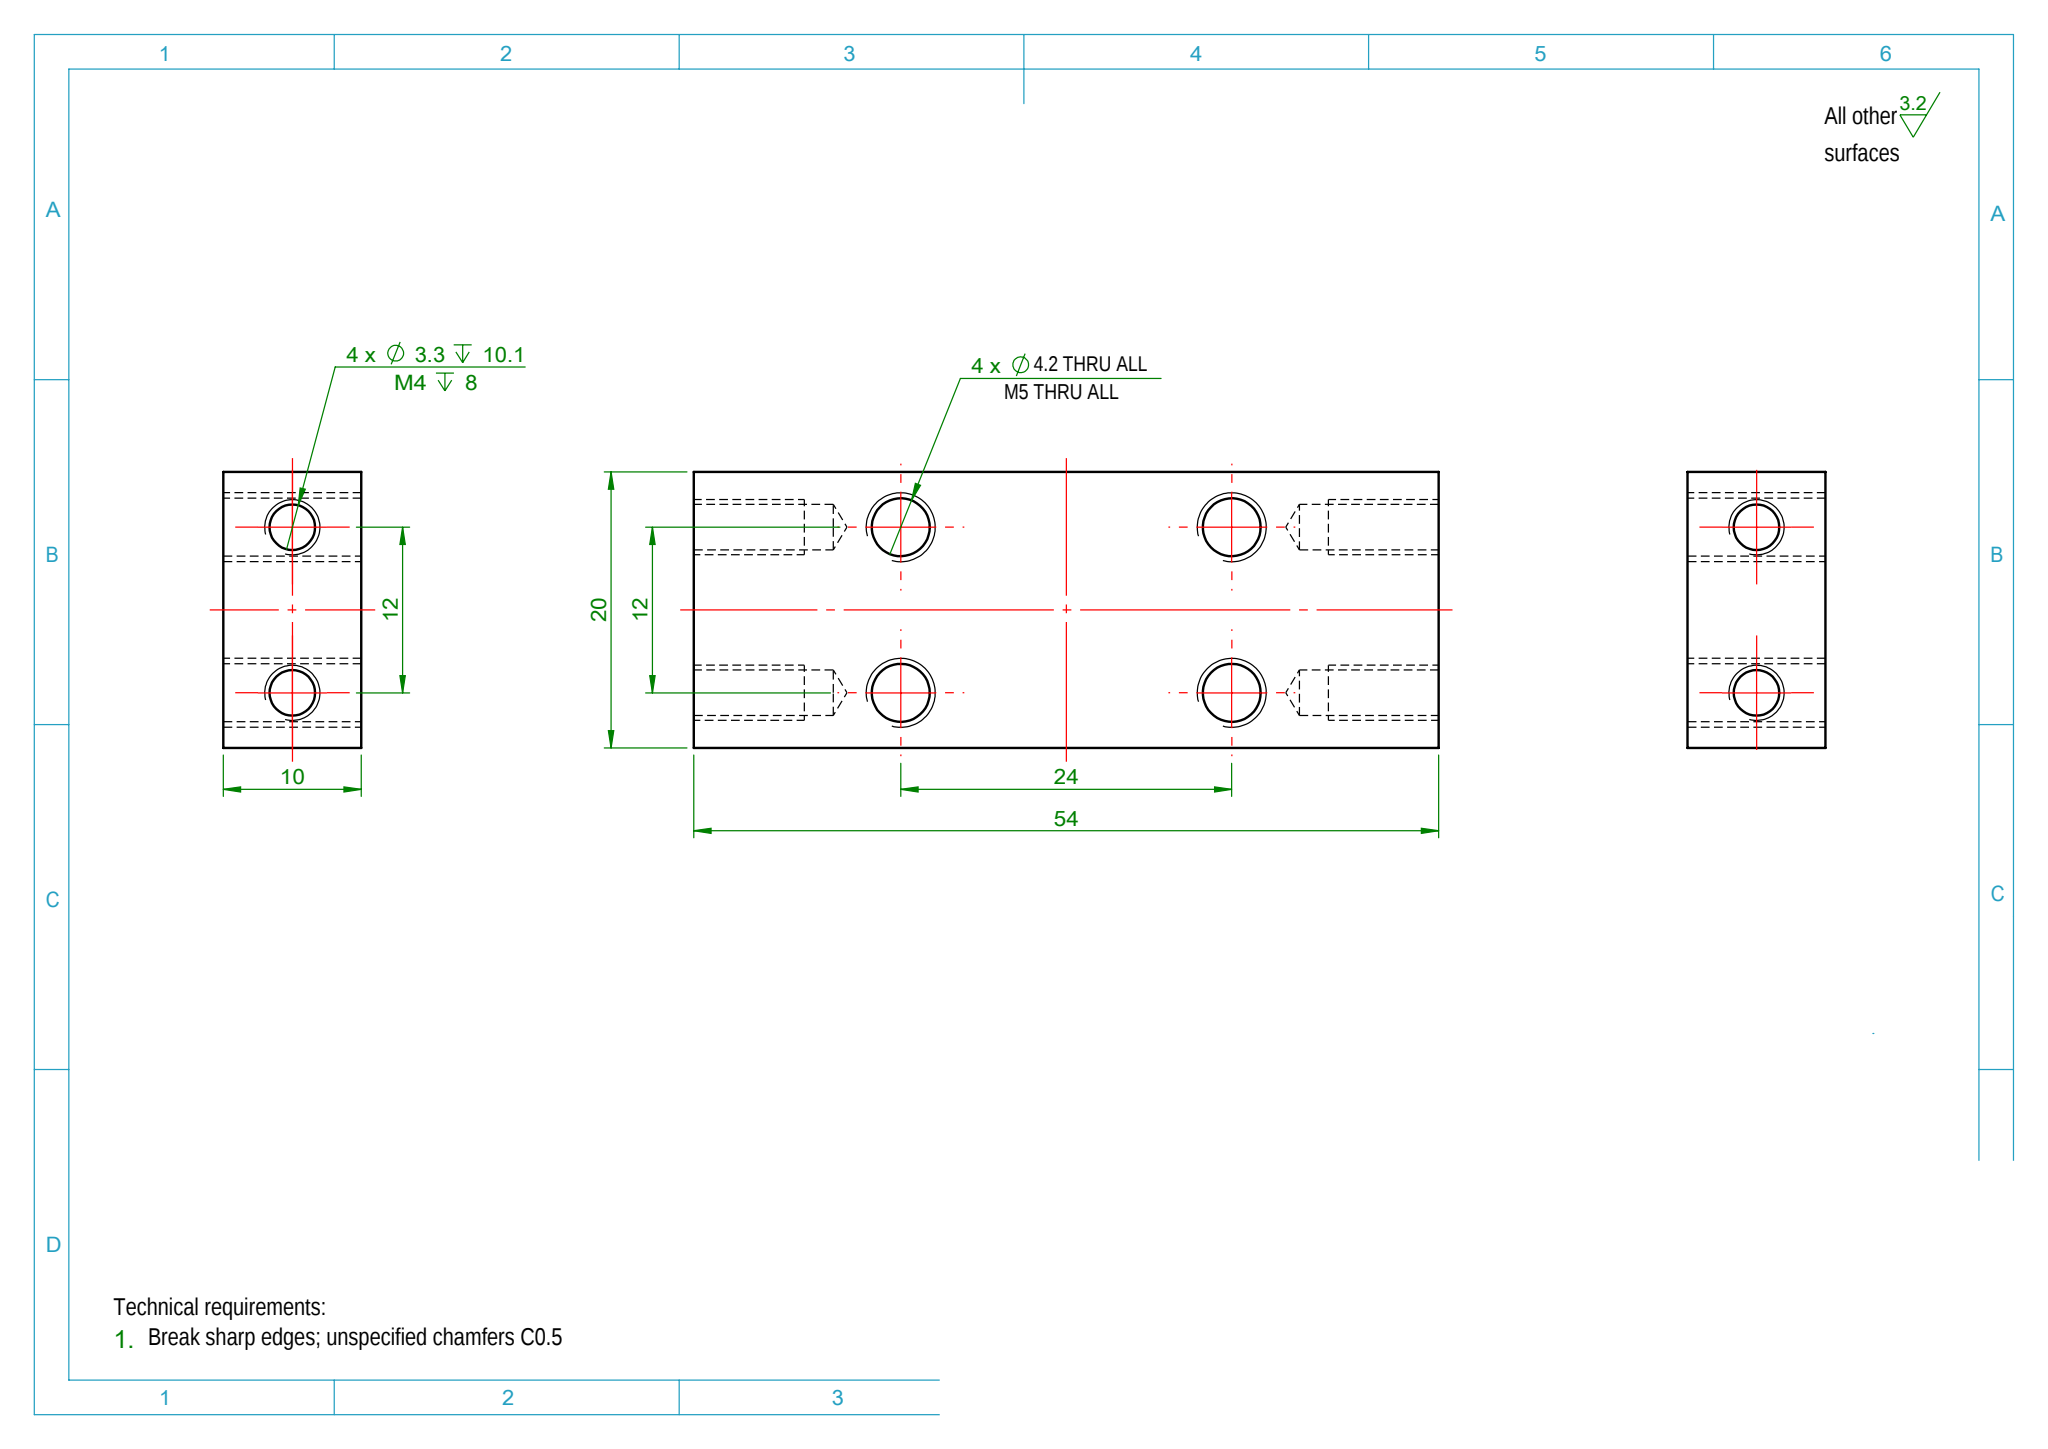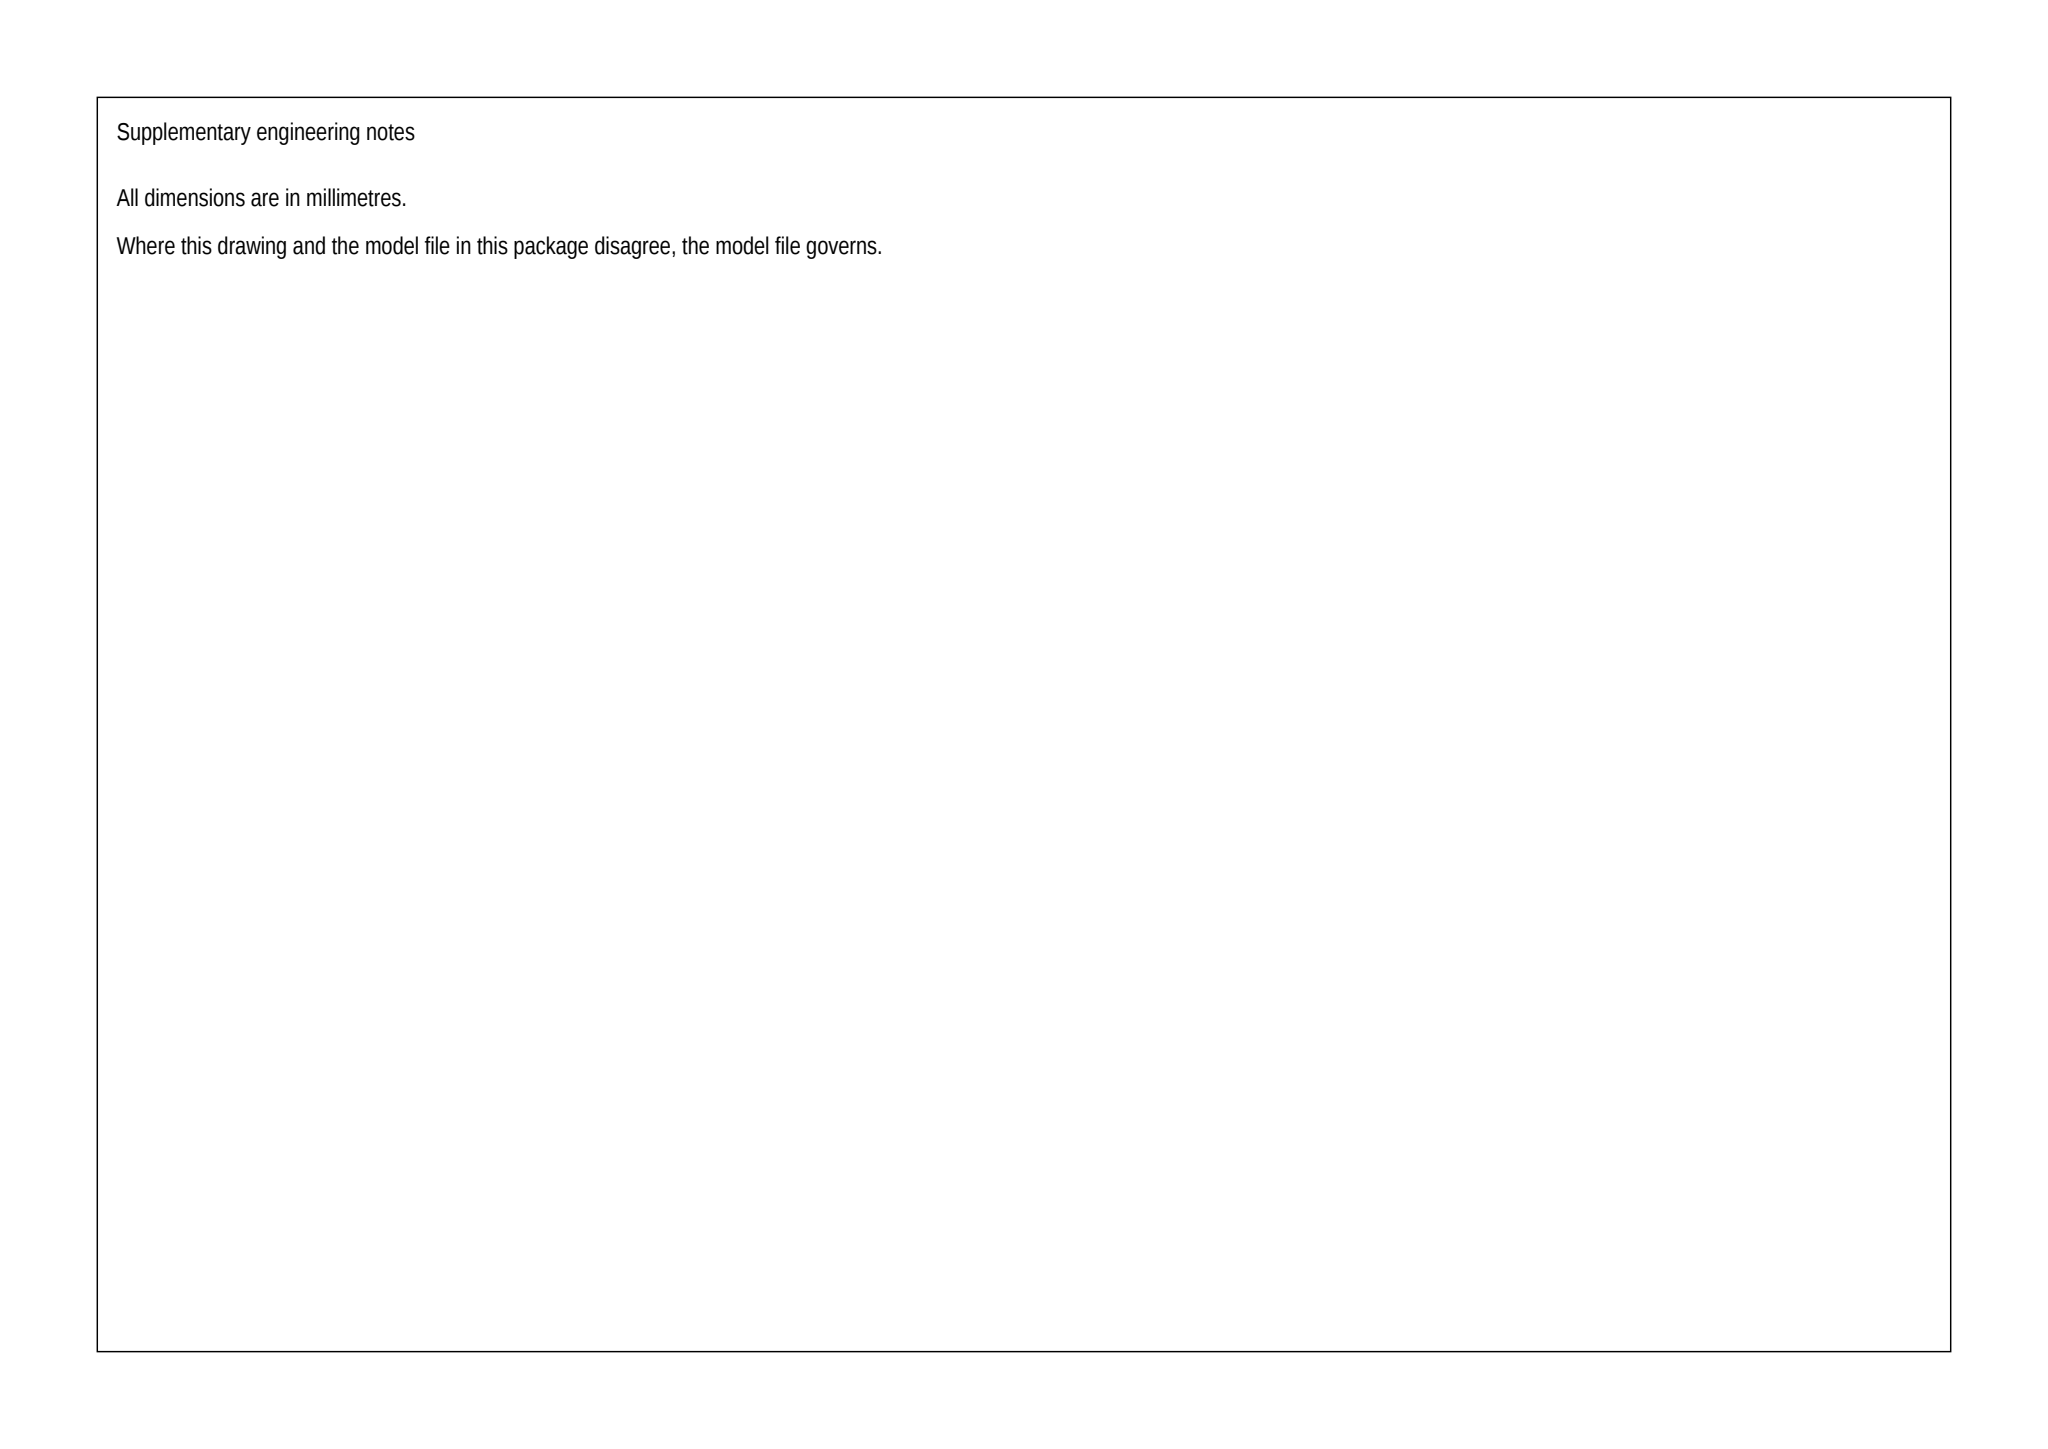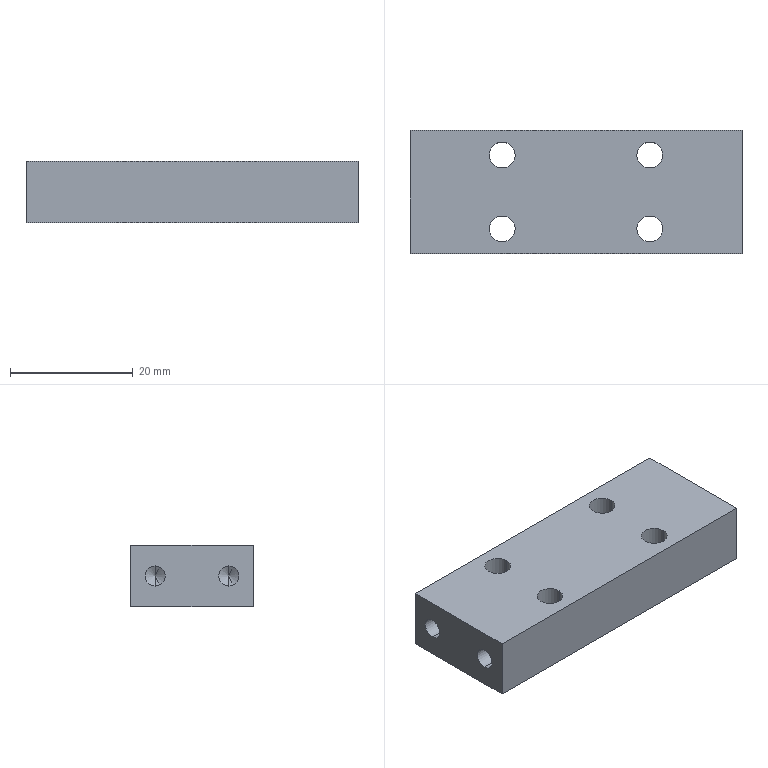Part | SolidWorks | mm | 1 solid | 30 faces | box 54 x 20 x 10 mm | volume 9889 mm3 | cylinder 16 | cone 8 | plane 6 | commonest cylinder face diameters 4.2 x8 3.3 x8
Drawing notes:
4X Ø4.2 THRU (through 10 thk plate), vertical axes; hole centers at X=15 and X=39 from left end face and Y=4 and Y=16 from bottom long edge. | from the solid: cylinders dia 4.2, axis z, length 10.0 at (15,4),(15,16),(39,4),(39,16); bbox_xyz 54x20x10
All dimensions in millimeters (mm) unless otherwise stated. | from the solid: STEP model units stated as mm; bbox_xyz [54.0, 20.0, 10.0]
build123d program:
from build123d import *

# Parameters (mm, degrees)
SKETCH1_W                  = 54
SKETCH1_H                  = 20
BOSS_EXTRUDE1_DEPTH        = 10
M4_TAPPED_HOLE1_AT_2_COUNT = 2
M4_TAPPED_HOLE1_AT_2_PITCH = 12
M5_TAPPED_HOLE1_D          = 4.2


with BuildPart() as part:
    # Sketch1 → Boss-Extrude1 (new body)
    with BuildSketch(Plane.XY):
        Rectangle(SKETCH1_W, SKETCH1_H)
    extrude(amount=BOSS_EXTRUDE1_DEPTH)

    # Sketch3 → M4 Tapped Hole1 (revolve, cut)
    with BuildSketch(Plane(origin=(-27, 6, 5), x_dir=(0, 0, 1), z_dir=(0, 1, 0))):
        Polygon((0, 0), (0, 11.091), (1.65, 10.1), (1.65, 0), align=None)
    m4_tapped_hole1 = revolve(axis=Axis((-33.35, 6, 5), (1, 0, 0)), mode=Mode.SUBTRACT)

    # M4 Tapped Hole1 at 2: M4 Tapped Hole1 ×2
    with Locations(*[(0, -i * M4_TAPPED_HOLE1_AT_2_PITCH, 0) for i in range(1, M4_TAPPED_HOLE1_AT_2_COUNT)]):
        add(m4_tapped_hole1, mode=Mode.SUBTRACT)

    # Mirror1: M4 Tapped Hole1 across plane
    add(m4_tapped_hole1.mirror(Plane(origin=(0, 0, 0), x_dir=(0, 0, 1), z_dir=(1, 0, 0))), mode=Mode.SUBTRACT)

    # Mirror1 copy 1 sketch → Mirror1 copy 1 (revolve, cut)
    with BuildSketch(Plane(origin=(27, -6, 5), x_dir=(0, 0, 1), z_dir=(0, 1, 0))):
        Polygon((0, 0), (0, -11.091), (1.65, -10.1), (1.65, 0), align=None)
    revolve(axis=Axis((33.35, -6, 5), (1, 0, 0)), mode=Mode.SUBTRACT)

    # M5 Tapped Hole1 (through all)
    with Locations(Plane.XY.offset(10)):
        with Locations((-12, 6), (-12, -6), (12, 6), (12, -6)):
            Hole(M5_TAPPED_HOLE1_D / 2)


solid = part.part
STEP:
#1=CARTESIAN_POINT('',(-14.1,6.,0.));
#2=VERTEX_POINT('',#1);
#3=CARTESIAN_POINT('',(-9.9,6.,0.));
#4=VERTEX_POINT('',#3);
#5=CARTESIAN_POINT('',(-12.,6.,0.));
#6=DIRECTION('',(0.,0.,1.));
#7=DIRECTION('',(1.,0.,0.));
#8=AXIS2_PLACEMENT_3D('',#5,#6,#7);
#9=CIRCLE('',#8,2.1);
#10=EDGE_CURVE('',#2,#4,#9,.T.);
#11=ORIENTED_EDGE('',*,*,#10,.F.);
#12=CARTESIAN_POINT('',(-14.1,6.,10.));
#13=VERTEX_POINT('',#12);
#14=CARTESIAN_POINT('',(-14.1,6.,10.));
#15=DIRECTION('',(0.,0.,1.));
#16=VECTOR('',#15,1000.);
#17=LINE('',#14,#16);
#18=EDGE_CURVE('',#2,#13,#17,.T.);
#19=ORIENTED_EDGE('',*,*,#18,.T.);
#20=CARTESIAN_POINT('',(-9.9,6.,10.));
#21=VERTEX_POINT('',#20);
#22=CARTESIAN_POINT('',(-12.,6.,10.));
#23=DIRECTION('',(0.,0.,1.));
#24=DIRECTION('',(1.,0.,0.));
#25=AXIS2_PLACEMENT_3D('',#22,#23,#24);
#26=CIRCLE('',#25,2.1);
#27=EDGE_CURVE('',#13,#21,#26,.T.);
#28=ORIENTED_EDGE('',*,*,#27,.T.);
#29=CARTESIAN_POINT('',(-9.9,6.,10.));
#30=DIRECTION('',(0.,0.,1.));
#31=VECTOR('',#30,1000.);
#32=LINE('',#29,#31);
#33=EDGE_CURVE('',#4,#21,#32,.T.);
#34=ORIENTED_EDGE('',*,*,#33,.F.);
#35=EDGE_LOOP('',(#11,#19,#28,#34));
#36=FACE_OUTER_BOUND('',#35,.T.);
#37=CARTESIAN_POINT('',(-12.,6.,10.));
#38=DIRECTION('',(0.,0.,1.));
#39=DIRECTION('',(1.,0.,0.));
#40=AXIS2_PLACEMENT_3D('',#37,#38,#39);
#41=CYLINDRICAL_SURFACE('',#40,2.1);
#42=ADVANCED_FACE('',(#36),#41,.F.);
#43=CARTESIAN_POINT('',(-14.1,-6.,0.));
#44=VERTEX_POINT('',#43);
#45=CARTESIAN_POINT('',(-9.9,-6.,0.));
#46=VERTEX_POINT('',#45);
#47=CARTESIAN_POINT('',(-12.,-6.,0.));
#48=DIRECTION('',(0.,0.,1.));
#49=DIRECTION('',(1.,0.,0.));
#50=AXIS2_PLACEMENT_3D('',#47,#48,#49);
#51=CIRCLE('',#50,2.1);
#52=EDGE_CURVE('',#44,#46,#51,.T.);
#53=ORIENTED_EDGE('',*,*,#52,.F.);
#54=CARTESIAN_POINT('',(-14.1,-6.,10.));
#55=VERTEX_POINT('',#54);
#56=CARTESIAN_POINT('',(-14.1,-6.,10.));
#57=DIRECTION('',(0.,0.,1.));
#58=VECTOR('',#57,1000.);
#59=LINE('',#56,#58);
#60=EDGE_CURVE('',#44,#55,#59,.T.);
#61=ORIENTED_EDGE('',*,*,#60,.T.);
#62=CARTESIAN_POINT('',(-9.9,-6.,10.));
#63=VERTEX_POINT('',#62);
#64=CARTESIAN_POINT('',(-12.,-6.,10.));
#65=DIRECTION('',(0.,0.,1.));
#66=DIRECTION('',(1.,0.,0.));
#67=AXIS2_PLACEMENT_3D('',#64,#65,#66);
#68=CIRCLE('',#67,2.1);
#69=EDGE_CURVE('',#55,#63,#68,.T.);
#70=ORIENTED_EDGE('',*,*,#69,.T.);
#71=CARTESIAN_POINT('',(-9.9,-6.,10.));
#72=DIRECTION('',(0.,0.,1.));
#73=VECTOR('',#72,1000.);
#74=LINE('',#71,#73);
#75=EDGE_CURVE('',#46,#63,#74,.T.);
#76=ORIENTED_EDGE('',*,*,#75,.F.);
#77=EDGE_LOOP('',(#53,#61,#70,#76));
#78=FACE_OUTER_BOUND('',#77,.T.);
#79=CARTESIAN_POINT('',(-12.,-6.,10.));
#80=DIRECTION('',(0.,0.,1.));
#81=DIRECTION('',(1.,0.,0.));
#82=AXIS2_PLACEMENT_3D('',#79,#80,#81);
#83=CYLINDRICAL_SURFACE('',#82,2.1);
#84=ADVANCED_FACE('',(#78),#83,.F.);
#85=CARTESIAN_POINT('',(9.9,6.,0.));
#86=VERTEX_POINT('',#85);
#87=CARTESIAN_POINT('',(14.1,6.,0.));
#88=VERTEX_POINT('',#87);
#89=CARTESIAN_POINT('',(12.,6.,0.));
#90=DIRECTION('',(0.,0.,1.));
#91=DIRECTION('',(1.,0.,0.));
#92=AXIS2_PLACEMENT_3D('',#89,#90,#91);
#93=CIRCLE('',#92,2.1);
#94=EDGE_CURVE('',#86,#88,#93,.T.);
#95=ORIENTED_EDGE('',*,*,#94,.F.);
#96=CARTESIAN_POINT('',(9.9,6.,10.));
#97=VERTEX_POINT('',#96);
#98=CARTESIAN_POINT('',(9.9,6.,10.));
#99=DIRECTION('',(0.,0.,1.));
#100=VECTOR('',#99,1000.);
#101=LINE('',#98,#100);
#102=EDGE_CURVE('',#86,#97,#101,.T.);
#103=ORIENTED_EDGE('',*,*,#102,.T.);
#104=CARTESIAN_POINT('',(14.1,6.,10.));
#105=VERTEX_POINT('',#104);
#106=CARTESIAN_POINT('',(12.,6.,10.));
#107=DIRECTION('',(0.,0.,1.));
#108=DIRECTION('',(1.,0.,0.));
#109=AXIS2_PLACEMENT_3D('',#106,#107,#108);
#110=CIRCLE('',#109,2.1);
#111=EDGE_CURVE('',#97,#105,#110,.T.);
#112=ORIENTED_EDGE('',*,*,#111,.T.);
#113=CARTESIAN_POINT('',(14.1,6.,10.));
#114=DIRECTION('',(0.,0.,1.));
#115=VECTOR('',#114,1000.);
#116=LINE('',#113,#115);
#117=EDGE_CURVE('',#88,#105,#116,.T.);
#118=ORIENTED_EDGE('',*,*,#117,.F.);
#119=EDGE_LOOP('',(#95,#103,#112,#118));
#120=FACE_OUTER_BOUND('',#119,.T.);
#121=CARTESIAN_POINT('',(12.,6.,10.));
#122=DIRECTION('',(0.,0.,1.));
#123=DIRECTION('',(1.,0.,0.));
#124=AXIS2_PLACEMENT_3D('',#121,#122,#123);
#125=CYLINDRICAL_SURFACE('',#124,2.1);
#126=ADVANCED_FACE('',(#120),#125,.F.);
#127=CARTESIAN_POINT('',(9.9,-6.,0.));
#128=VERTEX_POINT('',#127);
#129=CARTESIAN_POINT('',(14.1,-6.,0.));
#130=VERTEX_POINT('',#129);
#131=CARTESIAN_POINT('',(12.,-6.,0.));
#132=DIRECTION('',(0.,0.,1.));
#133=DIRECTION('',(1.,0.,0.));
#134=AXIS2_PLACEMENT_3D('',#131,#132,#133);
#135=CIRCLE('',#134,2.1);
#136=EDGE_CURVE('',#128,#130,#135,.T.);
#137=ORIENTED_EDGE('',*,*,#136,.F.);
#138=CARTESIAN_POINT('',(9.9,-6.,10.));
#139=VERTEX_POINT('',#138);
#140=CARTESIAN_POINT('',(9.9,-6.,10.));
#141=DIRECTION('',(0.,0.,1.));
#142=VECTOR('',#141,1000.);
#143=LINE('',#140,#142);
#144=EDGE_CURVE('',#128,#139,#143,.T.);
#145=ORIENTED_EDGE('',*,*,#144,.T.);
#146=CARTESIAN_POINT('',(14.1,-6.,10.));
#147=VERTEX_POINT('',#146);
#148=CARTESIAN_POINT('',(12.,-6.,10.));
#149=DIRECTION('',(0.,0.,1.));
#150=DIRECTION('',(1.,0.,0.));
#151=AXIS2_PLACEMENT_3D('',#148,#149,#150);
#152=CIRCLE('',#151,2.1);
#153=EDGE_CURVE('',#139,#147,#152,.T.);
#154=ORIENTED_EDGE('',*,*,#153,.T.);
#155=CARTESIAN_POINT('',(14.1,-6.,10.));
#156=DIRECTION('',(0.,0.,1.));
#157=VECTOR('',#156,1000.);
#158=LINE('',#155,#157);
#159=EDGE_CURVE('',#130,#147,#158,.T.);
#160=ORIENTED_EDGE('',*,*,#159,.F.);
#161=EDGE_LOOP('',(#137,#145,#154,#160));
#162=FACE_OUTER_BOUND('',#161,.T.);
#163=CARTESIAN_POINT('',(12.,-6.,10.));
#164=DIRECTION('',(0.,0.,1.));
#165=DIRECTION('',(1.,0.,0.));
#166=AXIS2_PLACEMENT_3D('',#163,#164,#165);
#167=CYLINDRICAL_SURFACE('',#166,2.1);
#168=ADVANCED_FACE('',(#162),#167,.F.);
#169=CARTESIAN_POINT('',(16.9,6.,6.65));
#170=VERTEX_POINT('',#169);
#171=CARTESIAN_POINT('',(16.9,6.,3.35));
#172=VERTEX_POINT('',#171);
#173=CARTESIAN_POINT('',(16.9,6.,5.));
#174=DIRECTION('',(1.,0.,0.));
#175=DIRECTION('',(0.,0.,-1.));
#176=AXIS2_PLACEMENT_3D('',#173,#174,#175);
#177=CIRCLE('',#176,1.65);
#178=EDGE_CURVE('',#170,#172,#177,.T.);
#179=ORIENTED_EDGE('',*,*,#178,.F.);
#180=CARTESIAN_POINT('',(27.,6.,6.65));
#181=VERTEX_POINT('',#180);
#182=CARTESIAN_POINT('',(27.,6.,6.65));
#183=DIRECTION('',(1.,0.,0.));
#184=VECTOR('',#183,1000.);
#185=LINE('',#182,#184);
#186=EDGE_CURVE('',#170,#181,#185,.T.);
#187=ORIENTED_EDGE('',*,*,#186,.T.);
#188=CARTESIAN_POINT('',(27.,6.,3.35));
#189=VERTEX_POINT('',#188);
#190=CARTESIAN_POINT('',(27.,6.,5.));
#191=DIRECTION('',(1.,0.,0.));
#192=DIRECTION('',(0.,0.,-1.));
#193=AXIS2_PLACEMENT_3D('',#190,#191,#192);
#194=CIRCLE('',#193,1.65);
#195=EDGE_CURVE('',#181,#189,#194,.T.);
#196=ORIENTED_EDGE('',*,*,#195,.T.);
#197=CARTESIAN_POINT('',(27.,6.,3.35));
#198=DIRECTION('',(1.,0.,0.));
#199=VECTOR('',#198,1000.);
#200=LINE('',#197,#199);
#201=EDGE_CURVE('',#172,#189,#200,.T.);
#202=ORIENTED_EDGE('',*,*,#201,.F.);
#203=EDGE_LOOP('',(#179,#187,#196,#202));
#204=FACE_OUTER_BOUND('',#203,.T.);
#205=CARTESIAN_POINT('',(27.,6.,5.));
#206=DIRECTION('',(1.,0.,0.));
#207=DIRECTION('',(0.,0.,-1.));
#208=AXIS2_PLACEMENT_3D('',#205,#206,#207);
#209=CYLINDRICAL_SURFACE('',#208,1.65);
#210=ADVANCED_FACE('',(#204),#209,.F.);
#211=CARTESIAN_POINT('',(15.909,6.,5.));
#212=VERTEX_POINT('',#211);
#213=CARTESIAN_POINT('',(16.9,6.,3.35));
#214=DIRECTION('',(0.515,0.,-0.8572));
#215=VECTOR('',#214,1000.);
#216=LINE('',#213,#215);
#217=EDGE_CURVE('',#212,#172,#216,.T.);
#218=ORIENTED_EDGE('',*,*,#217,.F.);
#219=CARTESIAN_POINT('',(16.9,6.,6.65));
#220=DIRECTION('',(0.515,0.,0.8572));
#221=VECTOR('',#220,1000.);
#222=LINE('',#219,#221);
#223=EDGE_CURVE('',#212,#170,#222,.T.);
#224=ORIENTED_EDGE('',*,*,#223,.T.);
#225=ORIENTED_EDGE('',*,*,#178,.T.);
#226=EDGE_LOOP('',(#218,#224,#225));
#227=FACE_OUTER_BOUND('',#226,.T.);
#228=CARTESIAN_POINT('',(16.9,6.,5.));
#229=DIRECTION('',(1.,0.,0.));
#230=DIRECTION('',(0.,0.,-1.));
#231=AXIS2_PLACEMENT_3D('',#228,#229,#230);
#232=CONICAL_SURFACE('',#231,1.65,1.03);
#233=ADVANCED_FACE('',(#227),#232,.F.);
#234=CARTESIAN_POINT('',(16.9,-6.,6.65));
#235=VERTEX_POINT('',#234);
#236=CARTESIAN_POINT('',(16.9,-6.,3.35));
#237=VERTEX_POINT('',#236);
#238=CARTESIAN_POINT('',(16.9,-6.,5.));
#239=DIRECTION('',(1.,0.,0.));
#240=DIRECTION('',(0.,0.,-1.));
#241=AXIS2_PLACEMENT_3D('',#238,#239,#240);
#242=CIRCLE('',#241,1.65);
#243=EDGE_CURVE('',#235,#237,#242,.T.);
#244=ORIENTED_EDGE('',*,*,#243,.F.);
#245=CARTESIAN_POINT('',(27.,-6.,6.65));
#246=VERTEX_POINT('',#245);
#247=CARTESIAN_POINT('',(27.,-6.,6.65));
#248=DIRECTION('',(1.,0.,0.));
#249=VECTOR('',#248,1000.);
#250=LINE('',#247,#249);
#251=EDGE_CURVE('',#235,#246,#250,.T.);
#252=ORIENTED_EDGE('',*,*,#251,.T.);
#253=CARTESIAN_POINT('',(27.,-6.,3.35));
#254=VERTEX_POINT('',#253);
#255=CARTESIAN_POINT('',(27.,-6.,5.));
#256=DIRECTION('',(1.,0.,0.));
#257=DIRECTION('',(0.,0.,-1.));
#258=AXIS2_PLACEMENT_3D('',#255,#256,#257);
#259=CIRCLE('',#258,1.65);
#260=EDGE_CURVE('',#246,#254,#259,.T.);
#261=ORIENTED_EDGE('',*,*,#260,.T.);
#262=CARTESIAN_POINT('',(27.,-6.,3.35));
#263=DIRECTION('',(1.,0.,0.));
#264=VECTOR('',#263,1000.);
#265=LINE('',#262,#264);
#266=EDGE_CURVE('',#237,#254,#265,.T.);
#267=ORIENTED_EDGE('',*,*,#266,.F.);
#268=EDGE_LOOP('',(#244,#252,#261,#267));
#269=FACE_OUTER_BOUND('',#268,.T.);
#270=CARTESIAN_POINT('',(27.,-6.,5.));
#271=DIRECTION('',(1.,0.,0.));
#272=DIRECTION('',(0.,0.,-1.));
#273=AXIS2_PLACEMENT_3D('',#270,#271,#272);
#274=CYLINDRICAL_SURFACE('',#273,1.65);
#275=ADVANCED_FACE('',(#269),#274,.F.);
#276=CARTESIAN_POINT('',(15.909,-6.,5.));
#277=VERTEX_POINT('',#276);
#278=CARTESIAN_POINT('',(16.9,-6.,3.35));
#279=DIRECTION('',(0.515,0.,-0.8572));
#280=VECTOR('',#279,1000.);
#281=LINE('',#278,#280);
#282=EDGE_CURVE('',#277,#237,#281,.T.);
#283=ORIENTED_EDGE('',*,*,#282,.F.);
#284=CARTESIAN_POINT('',(16.9,-6.,6.65));
#285=DIRECTION('',(0.515,0.,0.8572));
#286=VECTOR('',#285,1000.);
#287=LINE('',#284,#286);
#288=EDGE_CURVE('',#277,#235,#287,.T.);
#289=ORIENTED_EDGE('',*,*,#288,.T.);
#290=ORIENTED_EDGE('',*,*,#243,.T.);
#291=EDGE_LOOP('',(#283,#289,#290));
#292=FACE_OUTER_BOUND('',#291,.T.);
#293=CARTESIAN_POINT('',(16.9,-6.,5.));
#294=DIRECTION('',(1.,0.,0.));
#295=DIRECTION('',(0.,0.,-1.));
#296=AXIS2_PLACEMENT_3D('',#293,#294,#295);
#297=CONICAL_SURFACE('',#296,1.65,1.03);
#298=ADVANCED_FACE('',(#292),#297,.F.);
#299=CARTESIAN_POINT('',(-16.9,6.,3.35));
#300=VERTEX_POINT('',#299);
#301=CARTESIAN_POINT('',(-16.9,6.,6.65));
#302=VERTEX_POINT('',#301);
#303=CARTESIAN_POINT('',(-16.9,6.,5.));
#304=DIRECTION('',(-1.,0.,0.));
#305=DIRECTION('',(0.,0.,1.));
#306=AXIS2_PLACEMENT_3D('',#303,#304,#305);
#307=CIRCLE('',#306,1.65);
#308=EDGE_CURVE('',#300,#302,#307,.T.);
#309=ORIENTED_EDGE('',*,*,#308,.F.);
#310=CARTESIAN_POINT('',(-27.,6.,3.35));
#311=VERTEX_POINT('',#310);
#312=CARTESIAN_POINT('',(-27.,6.,3.35));
#313=DIRECTION('',(-1.,0.,0.));
#314=VECTOR('',#313,1000.);
#315=LINE('',#312,#314);
#316=EDGE_CURVE('',#300,#311,#315,.T.);
#317=ORIENTED_EDGE('',*,*,#316,.T.);
#318=CARTESIAN_POINT('',(-27.,6.,6.65));
#319=VERTEX_POINT('',#318);
#320=CARTESIAN_POINT('',(-27.,6.,5.));
#321=DIRECTION('',(-1.,0.,0.));
#322=DIRECTION('',(0.,0.,1.));
#323=AXIS2_PLACEMENT_3D('',#320,#321,#322);
#324=CIRCLE('',#323,1.65);
#325=EDGE_CURVE('',#311,#319,#324,.T.);
#326=ORIENTED_EDGE('',*,*,#325,.T.);
#327=CARTESIAN_POINT('',(-27.,6.,6.65));
#328=DIRECTION('',(-1.,0.,0.));
#329=VECTOR('',#328,1000.);
#330=LINE('',#327,#329);
#331=EDGE_CURVE('',#302,#319,#330,.T.);
#332=ORIENTED_EDGE('',*,*,#331,.F.);
#333=EDGE_LOOP('',(#309,#317,#326,#332));
#334=FACE_OUTER_BOUND('',#333,.T.);
#335=CARTESIAN_POINT('',(-27.,6.,5.));
#336=DIRECTION('',(-1.,0.,0.));
#337=DIRECTION('',(0.,0.,1.));
#338=AXIS2_PLACEMENT_3D('',#335,#336,#337);
#339=CYLINDRICAL_SURFACE('',#338,1.65);
#340=ADVANCED_FACE('',(#334),#339,.F.);
#341=CARTESIAN_POINT('',(-15.909,6.,5.));
#342=VERTEX_POINT('',#341);
#343=CARTESIAN_POINT('',(-16.9,6.,6.65));
#344=DIRECTION('',(-0.515,0.,0.8572));
#345=VECTOR('',#344,1000.);
#346=LINE('',#343,#345);
#347=EDGE_CURVE('',#342,#302,#346,.T.);
#348=ORIENTED_EDGE('',*,*,#347,.F.);
#349=CARTESIAN_POINT('',(-16.9,6.,3.35));
#350=DIRECTION('',(-0.515,0.,-0.8572));
#351=VECTOR('',#350,1000.);
#352=LINE('',#349,#351);
#353=EDGE_CURVE('',#342,#300,#352,.T.);
#354=ORIENTED_EDGE('',*,*,#353,.T.);
#355=ORIENTED_EDGE('',*,*,#308,.T.);
#356=EDGE_LOOP('',(#348,#354,#355));
#357=FACE_OUTER_BOUND('',#356,.T.);
#358=CARTESIAN_POINT('',(-16.9,6.,5.));
#359=DIRECTION('',(-1.,0.,0.));
#360=DIRECTION('',(0.,0.,1.));
#361=AXIS2_PLACEMENT_3D('',#358,#359,#360);
#362=CONICAL_SURFACE('',#361,1.65,1.03);
#363=ADVANCED_FACE('',(#357),#362,.F.);
#364=CARTESIAN_POINT('',(-16.9,-6.,3.35));
#365=VERTEX_POINT('',#364);
#366=CARTESIAN_POINT('',(-16.9,-6.,6.65));
#367=VERTEX_POINT('',#366);
#368=CARTESIAN_POINT('',(-16.9,-6.,5.));
#369=DIRECTION('',(-1.,0.,0.));
#370=DIRECTION('',(0.,0.,1.));
#371=AXIS2_PLACEMENT_3D('',#368,#369,#370);
#372=CIRCLE('',#371,1.65);
#373=EDGE_CURVE('',#365,#367,#372,.T.);
#374=ORIENTED_EDGE('',*,*,#373,.F.);
#375=CARTESIAN_POINT('',(-27.,-6.,3.35));
#376=VERTEX_POINT('',#375);
#377=CARTESIAN_POINT('',(-27.,-6.,3.35));
#378=DIRECTION('',(-1.,0.,0.));
#379=VECTOR('',#378,1000.);
#380=LINE('',#377,#379);
#381=EDGE_CURVE('',#365,#376,#380,.T.);
#382=ORIENTED_EDGE('',*,*,#381,.T.);
#383=CARTESIAN_POINT('',(-27.,-6.,6.65));
#384=VERTEX_POINT('',#383);
#385=CARTESIAN_POINT('',(-27.,-6.,5.));
#386=DIRECTION('',(-1.,0.,0.));
#387=DIRECTION('',(0.,0.,1.));
#388=AXIS2_PLACEMENT_3D('',#385,#386,#387);
#389=CIRCLE('',#388,1.65);
#390=EDGE_CURVE('',#376,#384,#389,.T.);
#391=ORIENTED_EDGE('',*,*,#390,.T.);
#392=CARTESIAN_POINT('',(-27.,-6.,6.65));
#393=DIRECTION('',(-1.,0.,0.));
#394=VECTOR('',#393,1000.);
#395=LINE('',#392,#394);
#396=EDGE_CURVE('',#367,#384,#395,.T.);
#397=ORIENTED_EDGE('',*,*,#396,.F.);
#398=EDGE_LOOP('',(#374,#382,#391,#397));
#399=FACE_OUTER_BOUND('',#398,.T.);
#400=CARTESIAN_POINT('',(-27.,-6.,5.));
#401=DIRECTION('',(-1.,0.,0.));
#402=DIRECTION('',(0.,0.,1.));
#403=AXIS2_PLACEMENT_3D('',#400,#401,#402);
#404=CYLINDRICAL_SURFACE('',#403,1.65);
#405=ADVANCED_FACE('',(#399),#404,.F.);
#406=CARTESIAN_POINT('',(-15.909,-6.,5.));
#407=VERTEX_POINT('',#406);
#408=CARTESIAN_POINT('',(-16.9,-6.,6.65));
#409=DIRECTION('',(-0.515,0.,0.8572));
#410=VECTOR('',#409,1000.);
#411=LINE('',#408,#410);
#412=EDGE_CURVE('',#407,#367,#411,.T.);
#413=ORIENTED_EDGE('',*,*,#412,.F.);
#414=CARTESIAN_POINT('',(-16.9,-6.,3.35));
#415=DIRECTION('',(-0.515,0.,-0.8572));
#416=VECTOR('',#415,1000.);
#417=LINE('',#414,#416);
#418=EDGE_CURVE('',#407,#365,#417,.T.);
#419=ORIENTED_EDGE('',*,*,#418,.T.);
#420=ORIENTED_EDGE('',*,*,#373,.T.);
#421=EDGE_LOOP('',(#413,#419,#420));
#422=FACE_OUTER_BOUND('',#421,.T.);
#423=CARTESIAN_POINT('',(-16.9,-6.,5.));
#424=DIRECTION('',(-1.,0.,0.));
#425=DIRECTION('',(0.,0.,1.));
#426=AXIS2_PLACEMENT_3D('',#423,#424,#425);
#427=CONICAL_SURFACE('',#426,1.65,1.03);
#428=ADVANCED_FACE('',(#422),#427,.F.);
#429=CARTESIAN_POINT('',(27.,6.,5.));
#430=DIRECTION('',(1.,0.,0.));
#431=DIRECTION('',(0.,0.,-1.));
#432=AXIS2_PLACEMENT_3D('',#429,#430,#431);
#433=CIRCLE('',#432,1.65);
#434=EDGE_CURVE('',#189,#181,#433,.T.);
#435=ORIENTED_EDGE('',*,*,#434,.F.);
#436=ORIENTED_EDGE('',*,*,#195,.F.);
#437=EDGE_LOOP('',(#435,#436));
#438=FACE_BOUND('',#437,.T.);
#439=CARTESIAN_POINT('',(27.,-6.,5.));
#440=DIRECTION('',(1.,0.,0.));
#441=DIRECTION('',(0.,0.,-1.));
#442=AXIS2_PLACEMENT_3D('',#439,#440,#441);
#443=CIRCLE('',#442,1.65);
#444=EDGE_CURVE('',#254,#246,#443,.T.);
#445=ORIENTED_EDGE('',*,*,#444,.F.);
#446=ORIENTED_EDGE('',*,*,#260,.F.);
#447=EDGE_LOOP('',(#445,#446));
#448=FACE_BOUND('',#447,.T.);
#449=CARTESIAN_POINT('',(27.,-10.,0.));
#450=VERTEX_POINT('',#449);
#451=CARTESIAN_POINT('',(27.,10.,0.));
#452=VERTEX_POINT('',#451);
#453=CARTESIAN_POINT('',(27.,10.,0.));
#454=DIRECTION('',(0.,1.,0.));
#455=VECTOR('',#454,1000.);
#456=LINE('',#453,#455);
#457=EDGE_CURVE('',#450,#452,#456,.T.);
#458=ORIENTED_EDGE('',*,*,#457,.T.);
#459=CARTESIAN_POINT('',(27.,10.,10.));
#460=VERTEX_POINT('',#459);
#461=CARTESIAN_POINT('',(27.,10.,10.));
#462=DIRECTION('',(0.,0.,-1.));
#463=VECTOR('',#462,1000.);
#464=LINE('',#461,#463);
#465=EDGE_CURVE('',#460,#452,#464,.T.);
#466=ORIENTED_EDGE('',*,*,#465,.F.);
#467=CARTESIAN_POINT('',(27.,-10.,10.));
#468=VERTEX_POINT('',#467);
#469=CARTESIAN_POINT('',(27.,10.,10.));
#470=DIRECTION('',(0.,1.,0.));
#471=VECTOR('',#470,1000.);
#472=LINE('',#469,#471);
#473=EDGE_CURVE('',#468,#460,#472,.T.);
#474=ORIENTED_EDGE('',*,*,#473,.F.);
#475=CARTESIAN_POINT('',(27.,-10.,10.));
#476=DIRECTION('',(0.,0.,-1.));
#477=VECTOR('',#476,1000.);
#478=LINE('',#475,#477);
#479=EDGE_CURVE('',#468,#450,#478,.T.);
#480=ORIENTED_EDGE('',*,*,#479,.T.);
#481=EDGE_LOOP('',(#458,#466,#474,#480));
#482=FACE_OUTER_BOUND('',#481,.T.);
#483=CARTESIAN_POINT('',(27.,10.,10.));
#484=DIRECTION('',(-1.,0.,0.));
#485=DIRECTION('',(0.,0.,1.));
#486=AXIS2_PLACEMENT_3D('',#483,#484,#485);
#487=PLANE('',#486);
#488=ADVANCED_FACE('',(#438,#448,#482),#487,.F.);
#489=CARTESIAN_POINT('',(-27.,10.,0.));
#490=VERTEX_POINT('',#489);
#491=CARTESIAN_POINT('',(-27.,10.,0.));
#492=DIRECTION('',(-1.,0.,0.));
#493=VECTOR('',#492,1000.);
#494=LINE('',#491,#493);
#495=EDGE_CURVE('',#452,#490,#494,.T.);
#496=ORIENTED_EDGE('',*,*,#495,.T.);
#497=CARTESIAN_POINT('',(-27.,10.,10.));
#498=VERTEX_POINT('',#497);
#499=CARTESIAN_POINT('',(-27.,10.,10.));
#500=DIRECTION('',(0.,0.,-1.));
#501=VECTOR('',#500,1000.);
#502=LINE('',#499,#501);
#503=EDGE_CURVE('',#498,#490,#502,.T.);
#504=ORIENTED_EDGE('',*,*,#503,.F.);
#505=CARTESIAN_POINT('',(-27.,10.,10.));
#506=DIRECTION('',(-1.,0.,0.));
#507=VECTOR('',#506,1000.);
#508=LINE('',#505,#507);
#509=EDGE_CURVE('',#460,#498,#508,.T.);
#510=ORIENTED_EDGE('',*,*,#509,.F.);
#511=ORIENTED_EDGE('',*,*,#465,.T.);
#512=EDGE_LOOP('',(#496,#504,#510,#511));
#513=FACE_OUTER_BOUND('',#512,.T.);
#514=CARTESIAN_POINT('',(-27.,10.,10.));
#515=DIRECTION('',(0.,-1.,0.));
#516=DIRECTION('',(0.,0.,-1.));
#517=AXIS2_PLACEMENT_3D('',#514,#515,#516);
#518=PLANE('',#517);
#519=ADVANCED_FACE('',(#513),#518,.F.);
#520=CARTESIAN_POINT('',(-27.,6.,5.));
#521=DIRECTION('',(-1.,0.,0.));
#522=DIRECTION('',(0.,0.,1.));
#523=AXIS2_PLACEMENT_3D('',#520,#521,#522);
#524=CIRCLE('',#523,1.65);
#525=EDGE_CURVE('',#319,#311,#524,.T.);
#526=ORIENTED_EDGE('',*,*,#525,.F.);
#527=ORIENTED_EDGE('',*,*,#325,.F.);
#528=EDGE_LOOP('',(#526,#527));
#529=FACE_BOUND('',#528,.T.);
#530=CARTESIAN_POINT('',(-27.,-6.,5.));
#531=DIRECTION('',(-1.,0.,0.));
#532=DIRECTION('',(0.,0.,1.));
#533=AXIS2_PLACEMENT_3D('',#530,#531,#532);
#534=CIRCLE('',#533,1.65);
#535=EDGE_CURVE('',#384,#376,#534,.T.);
#536=ORIENTED_EDGE('',*,*,#535,.F.);
#537=ORIENTED_EDGE('',*,*,#390,.F.);
#538=EDGE_LOOP('',(#536,#537));
#539=FACE_BOUND('',#538,.T.);
#540=CARTESIAN_POINT('',(-27.,-10.,0.));
#541=VERTEX_POINT('',#540);
#542=CARTESIAN_POINT('',(-27.,10.,0.));
#543=DIRECTION('',(0.,-1.,0.));
#544=VECTOR('',#543,1000.);
#545=LINE('',#542,#544);
#546=EDGE_CURVE('',#490,#541,#545,.T.);
#547=ORIENTED_EDGE('',*,*,#546,.T.);
#548=CARTESIAN_POINT('',(-27.,-10.,10.));
#549=VERTEX_POINT('',#548);
#550=CARTESIAN_POINT('',(-27.,-10.,10.));
#551=DIRECTION('',(0.,0.,-1.));
#552=VECTOR('',#551,1000.);
#553=LINE('',#550,#552);
#554=EDGE_CURVE('',#549,#541,#553,.T.);
#555=ORIENTED_EDGE('',*,*,#554,.F.);
#556=CARTESIAN_POINT('',(-27.,10.,10.));
#557=DIRECTION('',(0.,-1.,0.));
#558=VECTOR('',#557,1000.);
#559=LINE('',#556,#558);
#560=EDGE_CURVE('',#498,#549,#559,.T.);
#561=ORIENTED_EDGE('',*,*,#560,.F.);
#562=ORIENTED_EDGE('',*,*,#503,.T.);
#563=EDGE_LOOP('',(#547,#555,#561,#562));
#564=FACE_OUTER_BOUND('',#563,.T.);
#565=CARTESIAN_POINT('',(-27.,10.,10.));
#566=DIRECTION('',(1.,0.,0.));
#567=DIRECTION('',(0.,0.,-1.));
#568=AXIS2_PLACEMENT_3D('',#565,#566,#567);
#569=PLANE('',#568);
#570=ADVANCED_FACE('',(#529,#539,#564),#569,.F.);
#571=CARTESIAN_POINT('',(-27.,-10.,0.));
#572=DIRECTION('',(1.,0.,0.));
#573=VECTOR('',#572,1000.);
#574=LINE('',#571,#573);
#575=EDGE_CURVE('',#541,#450,#574,.T.);
#576=ORIENTED_EDGE('',*,*,#575,.T.);
#577=ORIENTED_EDGE('',*,*,#479,.F.);
#578=CARTESIAN_POINT('',(-27.,-10.,10.));
#579=DIRECTION('',(1.,0.,0.));
#580=VECTOR('',#579,1000.);
#581=LINE('',#578,#580);
#582=EDGE_CURVE('',#549,#468,#581,.T.);
#583=ORIENTED_EDGE('',*,*,#582,.F.);
#584=ORIENTED_EDGE('',*,*,#554,.T.);
#585=EDGE_LOOP('',(#576,#577,#583,#584));
#586=FACE_OUTER_BOUND('',#585,.T.);
#587=CARTESIAN_POINT('',(-27.,-10.,10.));
#588=DIRECTION('',(0.,1.,0.));
#589=DIRECTION('',(0.,0.,1.));
#590=AXIS2_PLACEMENT_3D('',#587,#588,#589);
#591=PLANE('',#590);
#592=ADVANCED_FACE('',(#586),#591,.F.);
#593=CARTESIAN_POINT('',(-12.,6.,10.));
#594=DIRECTION('',(0.,0.,1.));
#595=DIRECTION('',(1.,0.,0.));
#596=AXIS2_PLACEMENT_3D('',#593,#594,#595);
#597=CIRCLE('',#596,2.1);
#598=EDGE_CURVE('',#21,#13,#597,.T.);
#599=ORIENTED_EDGE('',*,*,#598,.F.);
#600=ORIENTED_EDGE('',*,*,#27,.F.);
#601=EDGE_LOOP('',(#599,#600));
#602=FACE_BOUND('',#601,.T.);
#603=CARTESIAN_POINT('',(-12.,-6.,10.));
#604=DIRECTION('',(0.,0.,1.));
#605=DIRECTION('',(1.,0.,0.));
#606=AXIS2_PLACEMENT_3D('',#603,#604,#605);
#607=CIRCLE('',#606,2.1);
#608=EDGE_CURVE('',#63,#55,#607,.T.);
#609=ORIENTED_EDGE('',*,*,#608,.F.);
#610=ORIENTED_EDGE('',*,*,#69,.F.);
#611=EDGE_LOOP('',(#609,#610));
#612=FACE_BOUND('',#611,.T.);
#613=CARTESIAN_POINT('',(12.,6.,10.));
#614=DIRECTION('',(0.,0.,1.));
#615=DIRECTION('',(1.,0.,0.));
#616=AXIS2_PLACEMENT_3D('',#613,#614,#615);
#617=CIRCLE('',#616,2.1);
#618=EDGE_CURVE('',#105,#97,#617,.T.);
#619=ORIENTED_EDGE('',*,*,#618,.F.);
#620=ORIENTED_EDGE('',*,*,#111,.F.);
#621=EDGE_LOOP('',(#619,#620));
#622=FACE_BOUND('',#621,.T.);
#623=CARTESIAN_POINT('',(12.,-6.,10.));
#624=DIRECTION('',(0.,0.,1.));
#625=DIRECTION('',(1.,0.,0.));
#626=AXIS2_PLACEMENT_3D('',#623,#624,#625);
#627=CIRCLE('',#626,2.1);
#628=EDGE_CURVE('',#147,#139,#627,.T.);
#629=ORIENTED_EDGE('',*,*,#628,.F.);
#630=ORIENTED_EDGE('',*,*,#153,.F.);
#631=EDGE_LOOP('',(#629,#630));
#632=FACE_BOUND('',#631,.T.);
#633=ORIENTED_EDGE('',*,*,#473,.T.);
#634=ORIENTED_EDGE('',*,*,#509,.T.);
#635=ORIENTED_EDGE('',*,*,#560,.T.);
#636=ORIENTED_EDGE('',*,*,#582,.T.);
#637=EDGE_LOOP('',(#633,#634,#635,#636));
#638=FACE_OUTER_BOUND('',#637,.T.);
#639=CARTESIAN_POINT('',(0.,0.,10.));
#640=DIRECTION('',(0.,0.,1.));
#641=DIRECTION('',(1.,0.,0.));
#642=AXIS2_PLACEMENT_3D('',#639,#640,#641);
#643=PLANE('',#642);
#644=ADVANCED_FACE('',(#602,#612,#622,#632,#638),#643,.T.);
#645=CARTESIAN_POINT('',(-12.,6.,0.));
#646=DIRECTION('',(0.,0.,1.));
#647=DIRECTION('',(1.,0.,0.));
#648=AXIS2_PLACEMENT_3D('',#645,#646,#647);
#649=CIRCLE('',#648,2.1);
#650=EDGE_CURVE('',#4,#2,#649,.T.);
#651=ORIENTED_EDGE('',*,*,#650,.T.);
#652=ORIENTED_EDGE('',*,*,#10,.T.);
#653=EDGE_LOOP('',(#651,#652));
#654=FACE_BOUND('',#653,.T.);
#655=CARTESIAN_POINT('',(-12.,-6.,0.));
#656=DIRECTION('',(0.,0.,1.));
#657=DIRECTION('',(1.,0.,0.));
#658=AXIS2_PLACEMENT_3D('',#655,#656,#657);
#659=CIRCLE('',#658,2.1);
#660=EDGE_CURVE('',#46,#44,#659,.T.);
#661=ORIENTED_EDGE('',*,*,#660,.T.);
#662=ORIENTED_EDGE('',*,*,#52,.T.);
#663=EDGE_LOOP('',(#661,#662));
#664=FACE_BOUND('',#663,.T.);
#665=CARTESIAN_POINT('',(12.,6.,0.));
#666=DIRECTION('',(0.,0.,1.));
#667=DIRECTION('',(1.,0.,0.));
#668=AXIS2_PLACEMENT_3D('',#665,#666,#667);
#669=CIRCLE('',#668,2.1);
#670=EDGE_CURVE('',#88,#86,#669,.T.);
#671=ORIENTED_EDGE('',*,*,#670,.T.);
#672=ORIENTED_EDGE('',*,*,#94,.T.);
#673=EDGE_LOOP('',(#671,#672));
#674=FACE_BOUND('',#673,.T.);
#675=CARTESIAN_POINT('',(12.,-6.,0.));
#676=DIRECTION('',(0.,0.,1.));
#677=DIRECTION('',(1.,0.,0.));
#678=AXIS2_PLACEMENT_3D('',#675,#676,#677);
#679=CIRCLE('',#678,2.1);
#680=EDGE_CURVE('',#130,#128,#679,.T.);
#681=ORIENTED_EDGE('',*,*,#680,.T.);
#682=ORIENTED_EDGE('',*,*,#136,.T.);
#683=EDGE_LOOP('',(#681,#682));
#684=FACE_BOUND('',#683,.T.);
#685=ORIENTED_EDGE('',*,*,#457,.F.);
#686=ORIENTED_EDGE('',*,*,#575,.F.);
#687=ORIENTED_EDGE('',*,*,#546,.F.);
#688=ORIENTED_EDGE('',*,*,#495,.F.);
#689=EDGE_LOOP('',(#685,#686,#687,#688));
#690=FACE_OUTER_BOUND('',#689,.T.);
#691=CARTESIAN_POINT('',(0.,0.,0.));
#692=DIRECTION('',(0.,0.,1.));
#693=DIRECTION('',(1.,0.,0.));
#694=AXIS2_PLACEMENT_3D('',#691,#692,#693);
#695=PLANE('',#694);
#696=ADVANCED_FACE('',(#654,#664,#674,#684,#690),#695,.F.);
#697=ORIENTED_EDGE('',*,*,#418,.F.);
#698=ORIENTED_EDGE('',*,*,#412,.T.);
#699=CARTESIAN_POINT('',(-16.9,-6.,5.));
#700=DIRECTION('',(-1.,0.,0.));
#701=DIRECTION('',(0.,0.,1.));
#702=AXIS2_PLACEMENT_3D('',#699,#700,#701);
#703=CIRCLE('',#702,1.65);
#704=EDGE_CURVE('',#367,#365,#703,.T.);
#705=ORIENTED_EDGE('',*,*,#704,.T.);
#706=EDGE_LOOP('',(#697,#698,#705));
#707=FACE_OUTER_BOUND('',#706,.T.);
#708=CARTESIAN_POINT('',(-16.9,-6.,5.));
#709=DIRECTION('',(-1.,0.,0.));
#710=DIRECTION('',(0.,0.,1.));
#711=AXIS2_PLACEMENT_3D('',#708,#709,#710);
#712=CONICAL_SURFACE('',#711,1.65,1.03);
#713=ADVANCED_FACE('',(#707),#712,.F.);
#714=ORIENTED_EDGE('',*,*,#381,.F.);
#715=ORIENTED_EDGE('',*,*,#704,.F.);
#716=ORIENTED_EDGE('',*,*,#396,.T.);
#717=ORIENTED_EDGE('',*,*,#535,.T.);
#718=EDGE_LOOP('',(#714,#715,#716,#717));
#719=FACE_OUTER_BOUND('',#718,.T.);
#720=CARTESIAN_POINT('',(-27.,-6.,5.));
#721=DIRECTION('',(-1.,0.,0.));
#722=DIRECTION('',(0.,0.,1.));
#723=AXIS2_PLACEMENT_3D('',#720,#721,#722);
#724=CYLINDRICAL_SURFACE('',#723,1.65);
#725=ADVANCED_FACE('',(#719),#724,.F.);
#726=ORIENTED_EDGE('',*,*,#353,.F.);
#727=ORIENTED_EDGE('',*,*,#347,.T.);
#728=CARTESIAN_POINT('',(-16.9,6.,5.));
#729=DIRECTION('',(-1.,0.,0.));
#730=DIRECTION('',(0.,0.,1.));
#731=AXIS2_PLACEMENT_3D('',#728,#729,#730);
#732=CIRCLE('',#731,1.65);
#733=EDGE_CURVE('',#302,#300,#732,.T.);
#734=ORIENTED_EDGE('',*,*,#733,.T.);
#735=EDGE_LOOP('',(#726,#727,#734));
#736=FACE_OUTER_BOUND('',#735,.T.);
#737=CARTESIAN_POINT('',(-16.9,6.,5.));
#738=DIRECTION('',(-1.,0.,0.));
#739=DIRECTION('',(0.,0.,1.));
#740=AXIS2_PLACEMENT_3D('',#737,#738,#739);
#741=CONICAL_SURFACE('',#740,1.65,1.03);
#742=ADVANCED_FACE('',(#736),#741,.F.);
#743=ORIENTED_EDGE('',*,*,#316,.F.);
#744=ORIENTED_EDGE('',*,*,#733,.F.);
#745=ORIENTED_EDGE('',*,*,#331,.T.);
#746=ORIENTED_EDGE('',*,*,#525,.T.);
#747=EDGE_LOOP('',(#743,#744,#745,#746));
#748=FACE_OUTER_BOUND('',#747,.T.);
#749=CARTESIAN_POINT('',(-27.,6.,5.));
#750=DIRECTION('',(-1.,0.,0.));
#751=DIRECTION('',(0.,0.,1.));
#752=AXIS2_PLACEMENT_3D('',#749,#750,#751);
#753=CYLINDRICAL_SURFACE('',#752,1.65);
#754=ADVANCED_FACE('',(#748),#753,.F.);
#755=ORIENTED_EDGE('',*,*,#288,.F.);
#756=ORIENTED_EDGE('',*,*,#282,.T.);
#757=CARTESIAN_POINT('',(16.9,-6.,5.));
#758=DIRECTION('',(1.,0.,0.));
#759=DIRECTION('',(0.,0.,-1.));
#760=AXIS2_PLACEMENT_3D('',#757,#758,#759);
#761=CIRCLE('',#760,1.65);
#762=EDGE_CURVE('',#237,#235,#761,.T.);
#763=ORIENTED_EDGE('',*,*,#762,.T.);
#764=EDGE_LOOP('',(#755,#756,#763));
#765=FACE_OUTER_BOUND('',#764,.T.);
#766=CARTESIAN_POINT('',(16.9,-6.,5.));
#767=DIRECTION('',(1.,0.,0.));
#768=DIRECTION('',(0.,0.,-1.));
#769=AXIS2_PLACEMENT_3D('',#766,#767,#768);
#770=CONICAL_SURFACE('',#769,1.65,1.03);
#771=ADVANCED_FACE('',(#765),#770,.F.);
#772=ORIENTED_EDGE('',*,*,#251,.F.);
#773=ORIENTED_EDGE('',*,*,#762,.F.);
#774=ORIENTED_EDGE('',*,*,#266,.T.);
#775=ORIENTED_EDGE('',*,*,#444,.T.);
#776=EDGE_LOOP('',(#772,#773,#774,#775));
#777=FACE_OUTER_BOUND('',#776,.T.);
#778=CARTESIAN_POINT('',(27.,-6.,5.));
#779=DIRECTION('',(1.,0.,0.));
#780=DIRECTION('',(0.,0.,-1.));
#781=AXIS2_PLACEMENT_3D('',#778,#779,#780);
#782=CYLINDRICAL_SURFACE('',#781,1.65);
#783=ADVANCED_FACE('',(#777),#782,.F.);
#784=ORIENTED_EDGE('',*,*,#223,.F.);
#785=ORIENTED_EDGE('',*,*,#217,.T.);
#786=CARTESIAN_POINT('',(16.9,6.,5.));
#787=DIRECTION('',(1.,0.,0.));
#788=DIRECTION('',(0.,0.,-1.));
#789=AXIS2_PLACEMENT_3D('',#786,#787,#788);
#790=CIRCLE('',#789,1.65);
#791=EDGE_CURVE('',#172,#170,#790,.T.);
#792=ORIENTED_EDGE('',*,*,#791,.T.);
#793=EDGE_LOOP('',(#784,#785,#792));
#794=FACE_OUTER_BOUND('',#793,.T.);
#795=CARTESIAN_POINT('',(16.9,6.,5.));
#796=DIRECTION('',(1.,0.,0.));
#797=DIRECTION('',(0.,0.,-1.));
#798=AXIS2_PLACEMENT_3D('',#795,#796,#797);
#799=CONICAL_SURFACE('',#798,1.65,1.03);
#800=ADVANCED_FACE('',(#794),#799,.F.);
#801=ORIENTED_EDGE('',*,*,#186,.F.);
#802=ORIENTED_EDGE('',*,*,#791,.F.);
#803=ORIENTED_EDGE('',*,*,#201,.T.);
#804=ORIENTED_EDGE('',*,*,#434,.T.);
#805=EDGE_LOOP('',(#801,#802,#803,#804));
#806=FACE_OUTER_BOUND('',#805,.T.);
#807=CARTESIAN_POINT('',(27.,6.,5.));
#808=DIRECTION('',(1.,0.,0.));
#809=DIRECTION('',(0.,0.,-1.));
#810=AXIS2_PLACEMENT_3D('',#807,#808,#809);
#811=CYLINDRICAL_SURFACE('',#810,1.65);
#812=ADVANCED_FACE('',(#806),#811,.F.);
#813=ORIENTED_EDGE('',*,*,#144,.F.);
#814=ORIENTED_EDGE('',*,*,#680,.F.);
#815=ORIENTED_EDGE('',*,*,#159,.T.);
#816=ORIENTED_EDGE('',*,*,#628,.T.);
#817=EDGE_LOOP('',(#813,#814,#815,#816));
#818=FACE_OUTER_BOUND('',#817,.T.);
#819=CARTESIAN_POINT('',(12.,-6.,10.));
#820=DIRECTION('',(0.,0.,1.));
#821=DIRECTION('',(1.,0.,0.));
#822=AXIS2_PLACEMENT_3D('',#819,#820,#821);
#823=CYLINDRICAL_SURFACE('',#822,2.1);
#824=ADVANCED_FACE('',(#818),#823,.F.);
#825=ORIENTED_EDGE('',*,*,#102,.F.);
#826=ORIENTED_EDGE('',*,*,#670,.F.);
#827=ORIENTED_EDGE('',*,*,#117,.T.);
#828=ORIENTED_EDGE('',*,*,#618,.T.);
#829=EDGE_LOOP('',(#825,#826,#827,#828));
#830=FACE_OUTER_BOUND('',#829,.T.);
#831=CARTESIAN_POINT('',(12.,6.,10.));
#832=DIRECTION('',(0.,0.,1.));
#833=DIRECTION('',(1.,0.,0.));
#834=AXIS2_PLACEMENT_3D('',#831,#832,#833);
#835=CYLINDRICAL_SURFACE('',#834,2.1);
#836=ADVANCED_FACE('',(#830),#835,.F.);
#837=ORIENTED_EDGE('',*,*,#60,.F.);
#838=ORIENTED_EDGE('',*,*,#660,.F.);
#839=ORIENTED_EDGE('',*,*,#75,.T.);
#840=ORIENTED_EDGE('',*,*,#608,.T.);
#841=EDGE_LOOP('',(#837,#838,#839,#840));
#842=FACE_OUTER_BOUND('',#841,.T.);
#843=CARTESIAN_POINT('',(-12.,-6.,10.));
#844=DIRECTION('',(0.,0.,1.));
#845=DIRECTION('',(1.,0.,0.));
#846=AXIS2_PLACEMENT_3D('',#843,#844,#845);
#847=CYLINDRICAL_SURFACE('',#846,2.1);
#848=ADVANCED_FACE('',(#842),#847,.F.);
#849=ORIENTED_EDGE('',*,*,#18,.F.);
#850=ORIENTED_EDGE('',*,*,#650,.F.);
#851=ORIENTED_EDGE('',*,*,#33,.T.);
#852=ORIENTED_EDGE('',*,*,#598,.T.);
#853=EDGE_LOOP('',(#849,#850,#851,#852));
#854=FACE_OUTER_BOUND('',#853,.T.);
#855=CARTESIAN_POINT('',(-12.,6.,10.));
#856=DIRECTION('',(0.,0.,1.));
#857=DIRECTION('',(1.,0.,0.));
#858=AXIS2_PLACEMENT_3D('',#855,#856,#857);
#859=CYLINDRICAL_SURFACE('',#858,2.1);
#860=ADVANCED_FACE('',(#854),#859,.F.);
#861=CLOSED_SHELL('',(#42,#84,#126,#168,#210,#233,#275,#298,#340,#363,#405,#428,#488,#519,#570,#592,#644,#696,#713,#725,#742,#754,#771,#783,#800,#812,#824,#836,#848,#860));
#862=MANIFOLD_SOLID_BREP('',#861);
#863=CARTESIAN_POINT('',(0.,0.,0.));
#864=DIRECTION('',(0.,0.,1.));
#865=DIRECTION('',(1.,0.,0.));
#866=AXIS2_PLACEMENT_3D('',#863,#864,#865);
#867=(LENGTH_UNIT()NAMED_UNIT(*)SI_UNIT(.MILLI.,.METRE.));
#868=UNCERTAINTY_MEASURE_WITH_UNIT(LENGTH_MEASURE(0.00001),#867,'','');
#869=(NAMED_UNIT(*)PLANE_ANGLE_UNIT()SI_UNIT($,.RADIAN.));
#870=(NAMED_UNIT(*)SI_UNIT($,.STERADIAN.)SOLID_ANGLE_UNIT());
#871=(GEOMETRIC_REPRESENTATION_CONTEXT(3)GLOBAL_UNCERTAINTY_ASSIGNED_CONTEXT((#868))GLOBAL_UNIT_ASSIGNED_CONTEXT((#867,#869,#870))REPRESENTATION_CONTEXT('',''));
#872=ADVANCED_BREP_SHAPE_REPRESENTATION('',(#862,#866),#871);